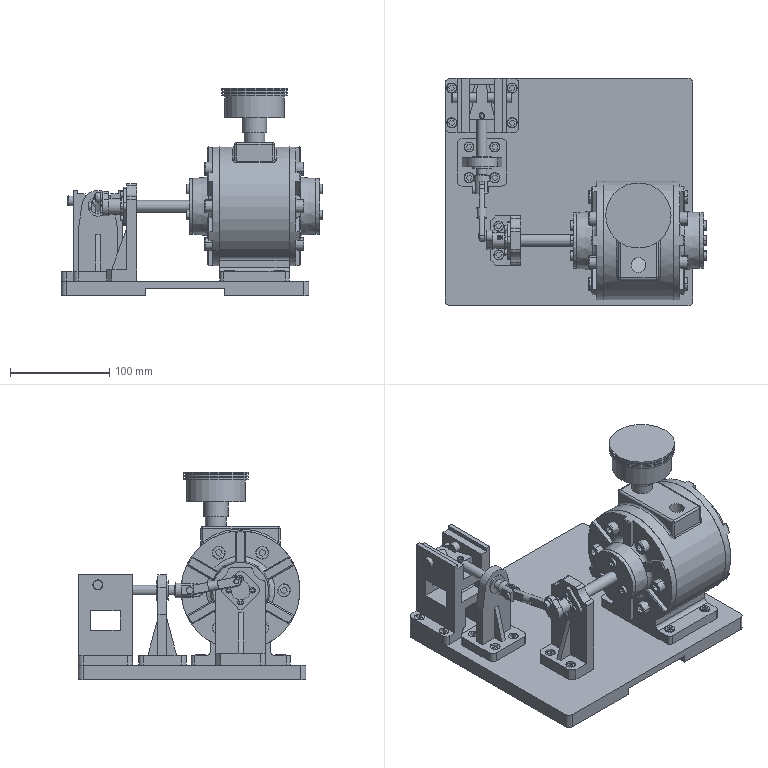Assembly | NX | mm | 57 component files | 57 solids | 1471 faces | box 264 x 230 x 210 mm | volume 1858746 mm3 | plane 707 | cylinder 372 | cone 206 | torus 175 | sphere 6 | spline 5 | commonest cylinder face diameters 10 x80 6 x68 8 x59 13 x24 4 x21 3 x18 6.6 x14 5 x14
Bill of materials:
unnamed part 1 | 1 |  | Cylindrical pin with chamfered ends and a flat-sided rectangular key along one side; a rectangular cutout in the key leaves a short tab near one end and a longer section near the other end.
unnamed part 2 | 1 |  | Stepped coaxial round body: a large flat-topped cylindrical head with three narrow circumferential grooves near the top face, then two progressively smaller cylindrical steps below.
unnamed part 3 | 1 |  | Long, flat bar with fully rounded (stadium-shaped) ends, flat top and bottom faces, and small edge chamfers or rounds.
unnamed part 4 | 12 |  | Stepped cylindrical pin: a short, larger-diameter head with a slightly rounded outer edge, and a smaller coaxial plain shank with a chamfered tip and a small fillet at the shoulder.
unnamed part 5 | 1 |  | Rectangular block with a diagonal, angled channel or slot cut across the top, a stepped lower ledge along one edge, a round through-bore in one side face, and a small countersunk or counterbored hole on the top face.
unnamed part 6 | 6 |  | Cylindrical-head fastener shape with a hexagonal socket in the head end, a plain cylindrical shank, and a chamfered tip.
unnamed part 7 | 1 |  | Long round shaft with a forked (clevis-style) end at one end: two parallel prongs with a cross hole through them. Next to the fork is a larger collar, then a long main shaft that steps down to a smaller-diameter end with a small cross hole.
unnamed part 8 | 2 |  | Thin flat circular disc with a large central hole and three smaller holes evenly spaced on a circle around it.
unnamed part 9 | 4 |  | Stepped cylindrical pin: a larger cylindrical head with a slightly rounded outer edge and a smaller, longer coaxial plain shank with a chamfered tip.
unnamed part 10 | 1 |  | Bracket with a rectangular base plate (rounded corners, four corner through-holes) and a single upright lug. The lug has a rounded top, a cross hole with a raised boss, and tapered triangular gussets on both sides.
unnamed part 11 | 1 |  | Short cylindrical-head fastener shape with a hexagonal socket in the head, a short plain shank, and a chamfered tip.
unnamed part 12 | 1 |  | Cylindrical pin with chamfered ends and a flat-bottomed rectangular key along one side; a rectangular cutout leaves a longer key section at one end and a short tab at the other. It looks like a mirrored version of the similar part.
unnamed part 13 | 1 |  | Headed cylindrical pin: a short larger-diameter cylindrical head, a long plain shank, and a narrow circumferential groove near the far end of the shank.
unnamed part 14 | 1 |  | Radial bladed rotor: a cylindrical hub with six curved, swept rectangular blades. The hub has a central bore with a single keyway notch.
unnamed part 15 | 1 |  | H-shaped bracket or frame: two parallel upright plates joined by cross members, set on a rectangular base with rounded corners. The base has four through holes and a central relief cut out underneath.
unnamed part 16 | 1 |  | Flat link bar with rounded ends: an elongated bar with a through hole at each end and a short cylindrical boss across the middle, perpendicular to the bar's flat faces.
unnamed part 17 | 1 |  | Crank-like body: a teardrop-shaped plate (lobe) with a hollow cylindrical sleeve on one side and a small stepped pin on the other side, offset from the sleeve.
unnamed part 18 | 1 |  | L-shaped mounting bracket: a tall upright plate with a curved notched top and a short base foot with two through holes. The upright carries a central hole and a four-hole pattern around it.
unnamed part 19 | 1 |  | Cylindrical housing on a footed base: an annular body with a large through bore, six holes on a bolt circle on the face, a rectangular pad on top with a hole and a small tubular boss, and a flat base foot with four holes.
unnamed part 20 | 1 |  | Flat rectangular plate with small rounded corners, pierced by sixteen small through holes in several clusters. A shallow rectangular recess or step runs across part of the underside.
unnamed part 21 | 1 |  | Long stepped shaft: a larger-diameter main section, a longer reduced-diameter section, and a short smaller end journal at each end. There is a small cross hole near one end.
unnamed part 22 | 2 |  | Circular flanged hub: a flat disc with a raised central hub that has a center bore. The disc has six outer through holes and six radial rib or groove features, and the hub face has three smaller holes.
unnamed part 23 | 14 |  | Cap-head fastener shape: a cylindrical head with a hexagonal socket recess and a plain cylindrical shank with a chamfered tip.
Mates:
1. fix | Base 1 component
2. concentric | Base 1 edge | Work_Table 1 edge
3. parallel | Work_Table 1 face | Base 1 face
4. touch align | Work_Table 1 face | Slider 1 face
5. center | Slider 1 face | Slider 1 face | Work_Table 1 face | Work_Table 1 face
6. parallel | Guide_Pillar_A 1 face | Base 1 face
7. touch align | Guide_Pillar_A 1 face | Work_Table 1 face
8. touch align | Guide_Pillar_A 1 face | Slider 1 face
9. concentric | Base 1 edge | Bracket_B 1 edge
10. parallel | Bracket_B 1 face | Base 1 face
11. concentric | Base 1 edge | Bracket_A 1 edge
12. parallel | Bracket_A 1 face | Base 1 face
13. concentric | Base 1 edge | Housing 1 edge
14. parallel | Housing 1 face | Base 1 face
15. concentric | Housing 1 edge | Front_Casing_Cover 2 edge
16. concentric | Front_Casing_Cover 2 edge | Housing 1 edge
17. concentric | Front_Casing_Cover 1 edge | Housing 1 edge
18. concentric | Front_Casing_Cover 1 edge | Housing 1 edge
19. concentric | Front_Casing_Cover 2 edge | Front_End_Cover 2 edge
20. concentric | Front_End_Cover 2 edge | Front_Casing_Cover 2 edge
21. concentric | Front_Casing_Cover 1 edge | Front_End_Cover 1 edge
22. concentric | Front_End_Cover 1 edge | Front_Casing_Cover 1 edge
23. touch align | Shaft 1 face | Front_Casing_Cover 1 face
24. center | Shaft 1 face | Shaft 1 face | Front_End_Cover 1 face | Front_End_Cover 2 face
25. touch align | Crank 1 face | Shaft 1 face
26. touch align | Crank 1 face | Shaft 1 face
27. touch align | Push_Rod 1 face | Bracket_B 1 face
28. touch align | Push_Rod 1 face | Slider 1 face
29. touch align | Connecting_Rod 1 face | Push_Rod 1 face
30. center | Connecting_Rod 1 face | Connecting_Rod 1 face | Push_Rod 1 face | Push_Rod 1 face
31. touch align | Connecting_Rod 1 face | Crank 1 face
32. concentric | Air_Pump 1 edge | Housing 1 edge
33. concentric | Pin 1 edge | Push_Rod 1 edge
34. concentric | Hex_Socket_Cap_Screw_M6x16 14 edge | Work_Table 1 edge
35. concentric | Hex_Socket_Cap_Screw_M6x16 13 edge | Work_Table 1 edge
36. concentric | Hex_Socket_Cap_Screw_M6x16 12 edge | Work_Table 1 edge
37. concentric | Hex_Socket_Cap_Screw_M6x16 11 edge | Work_Table 1 edge
38. concentric | Hex_Socket_Cap_Screw_M6x16 10 edge | Bracket_B 1 edge
39. concentric | Hex_Socket_Cap_Screw_M6x16 9 edge | Bracket_A 1 edge
40. concentric | Hex_Socket_Cap_Screw_M6x16 8 edge | Bracket_A 1 edge
41. concentric | Hex_Socket_Cap_Screw_M6x16 7 edge | Housing 1 edge
42. concentric | Hex_Socket_Cap_Screw_M6x16 6 edge | Bracket_B 1 edge
43. concentric | Hex_Socket_Cap_Screw_M6x16 5 edge | Bracket_B 1 edge
44. concentric | Hex_Socket_Cap_Screw_M6x16 4 edge | Bracket_B 1 edge
45. concentric | Hex_Socket_Cap_Screw_M6x16 3 edge | Housing 1 edge
46. concentric | Hex_Socket_Cap_Screw_M6x16 2 edge | Housing 1 edge
47. concentric | Hex_Socket_Cap_Screw_M6x16 1 edge | Housing 1 edge
48. concentric | Hex_Socket_Cap_Screw_M8x12 12 edge | Front_Casing_Cover 1 edge
49. bond | Front_Casing_Cover 1 component | assembly component
50. bond | Hex_Socket_Cap_Screw_M8x12 12 component | assembly component
51. bond | Hex_Socket_Cap_Screw_M8x12 11 component | assembly component
52. bond | Hex_Socket_Cap_Screw_M8x12 10 component | assembly component
53. bond | Hex_Socket_Cap_Screw_M8x12 9 component | assembly component
54. bond | Hex_Socket_Cap_Screw_M8x12 8 component | assembly component
55. bond | Hex_Socket_Cap_Screw_M8x12 7 component | assembly component
56. circular | assembly datumaxis | assembly cartesiancoordinatesystem | assembly cartesiancoordinatesystem | assembly cartesiancoordinatesystem | assembly cartesiancoordinatesystem | assembly cartesiancoordinatesystem | assembly cartesiancoordinatesystem
57. concentric | Hex_Socket_Cap_Screw_M8x12 6 edge | Front_Casing_Cover 2 edge
58. bond | Front_Casing_Cover 2 component | assembly component
59. bond | Hex_Socket_Cap_Screw_M8x12 6 component | assembly component
60. bond | Hex_Socket_Cap_Screw_M8x12 5 component | assembly component
61. bond | Hex_Socket_Cap_Screw_M8x12 4 component | assembly component
62. bond | Hex_Socket_Cap_Screw_M8x12 3 component | assembly component
63. bond | Hex_Socket_Cap_Screw_M8x12 2 component | assembly component
64. bond | Hex_Socket_Cap_Screw_M8x12 1 component | assembly component
65. circular | assembly datumaxis | assembly cartesiancoordinatesystem | assembly cartesiancoordinatesystem | assembly cartesiancoordinatesystem | assembly cartesiancoordinatesystem | assembly cartesiancoordinatesystem | assembly cartesiancoordinatesystem
66. touch align | Guide_Pillar_B 1 face | Work_Table 1 face
67. parallel | Guide_Pillar_B 1 face | Work_Table 1 face
68. touch align | Guide_Pillar_B 1 face | Slider 1 face
69. concentric | GB_T_70_1_2008_Hex_Socket_Cap_Screw_M6x16 6 edge | Front_End_Cover 2 edge
70. bond | Front_End_Cover 2 component | assembly component
71. bond | GB_T_70_1_2008_Hex_Socket_Cap_Screw_M6x16 6 component | assembly component
72. bond | GB_T_70_1_2008_Hex_Socket_Cap_Screw_M6x16 5 component | assembly component
73. bond | GB_T_70_1_2008_Hex_Socket_Cap_Screw_M6x16 4 component | assembly component
74. circular | assembly datumaxis | assembly cartesiancoordinatesystem | assembly cartesiancoordinatesystem | assembly cartesiancoordinatesystem
75. concentric | GB_T_70_1_2008_Hex_Socket_Cap_Screw_M3x8 4 edge | Bracket_A 1 edge
76. bond | Crank 1 component | assembly component
77. bond | GB_T_70_1_2008_Hex_Socket_Cap_Screw_M3x8 4 component | assembly component
78. bond | GB_T_70_1_2008_Hex_Socket_Cap_Screw_M3x8 3 component | assembly component
79. bond | GB_T_70_1_2008_Hex_Socket_Cap_Screw_M3x8 2 component | assembly component
80. circular | assembly datumaxis | assembly cartesiancoordinatesystem | assembly cartesiancoordinatesystem | assembly cartesiancoordinatesystem | assembly cartesiancoordinatesystem
81. bond | GB_T_70_1_2008_Hex_Socket_Cap_Screw_M3x8 1 component | assembly component
82. concentric | GB_T_70_1_2008_Hex_Socket_Cap_Screw_M6x16 3 edge | Front_End_Cover 1 edge
83. bond | Front_End_Cover 1 component | assembly component
84. bond | GB_T_70_1_2008_Hex_Socket_Cap_Screw_M6x16 3 component | assembly component
85. bond | GB_T_70_1_2008_Hex_Socket_Cap_Screw_M6x16 2 component | assembly component
86. bond | GB_T_70_1_2008_Hex_Socket_Cap_Screw_M6x16 1 component | assembly component
87. circular | assembly datumaxis | assembly cartesiancoordinatesystem | assembly cartesiancoordinatesystem | assembly cartesiancoordinatesystem
88. touch align | Flywheel 1 face | Shaft 1 face
89. parallel | Shaft 1 face | Flywheel 1 face
90. center | Flywheel 1 face | Flywheel 1 face | Front_Casing_Cover 2 face | Front_Casing_Cover 1 face
91. concentric | GB_T_70_1_2008_Hex_Socket_Cap_Screw_M3x5 1 edge | Slider 1 edge
92. concentric | Key 1 arc | Shaft 1 edge
93. parallel | Key 1 face | Shaft 1 face